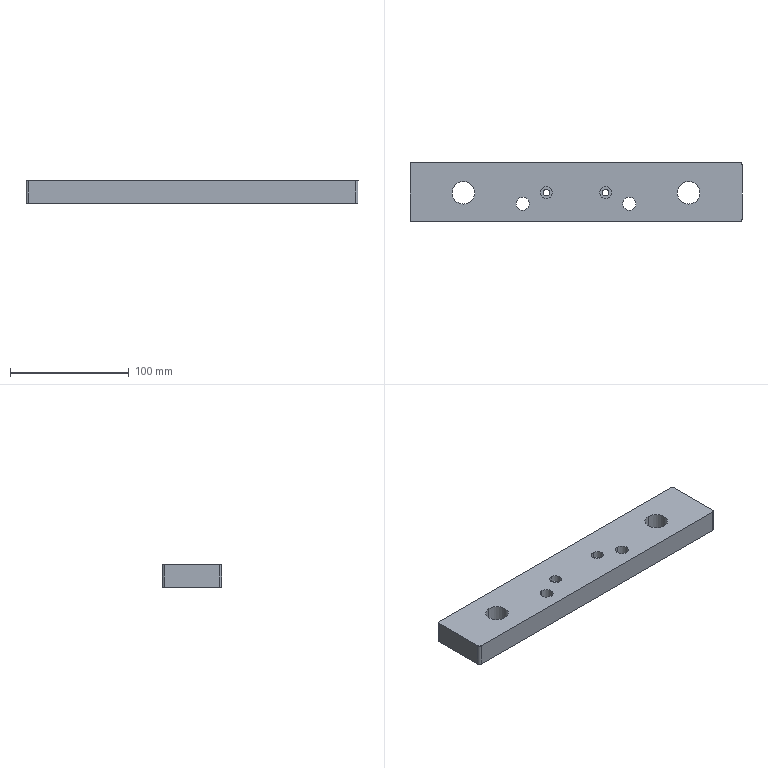Component | SolidWorks | 2SZT-2-001-3 | 1 solid | 33 faces | box 280 x 50 x 19.01 mm | volume 247242 mm3 | cylinder 20 | plane 13 | commonest cylinder face diameters 11 x4 10 x4 5.5 x4 19.02 x4 4 x4
build123d program:
from build123d import *

# Parameters (mm, degrees)
SKETCH1_W                                            = 280
SKETCH1_H                                            = 50
BOSS_EXTRUDE1_DEPTH                                  = 19
FILLET1_R                                            = 2
FILLET2_R                                            = 2
FILLET3_R                                            = 2
FILLET4_R                                            = 2
SKETCH11_W                                           = 62
SKETCH11_H                                           = 23
CUT_EXTRUDE2_DEPTH                                   = 2
F_10_0_10_DIAMETER_HOLE1_D                           = 19.02
F_10_0_10_DIAMETER_HOLE1_DEPTH                       = 70
F_10_0_10_DIAMETER_HOLE1_TIP                         = 5.714
HOLE_SIZE_ACCORDING_TO_THE_TYPE_OF_HEXAG_D           = 5.5
HOLE_SIZE_ACCORDING_TO_THE_TYPE_OF_HEXAG_CBORE_D     = 10
HOLE_SIZE_ACCORDING_TO_THE_TYPE_OF_HEXAG_CBORE_DEPTH = 5.7
F_11_0_11_DIAMETER_HOLE1_D                           = 11
F_11_0_11_DIAMETER_HOLE1_DEPTH                       = 20
F_11_0_11_DIAMETER_HOLE1_TIP                         = 3.305


with BuildPart() as part:
    # Sketch1 → Boss-Extrude1 (new body)
    with BuildSketch(Plane(origin=(0, 117.1, 0), x_dir=(-1, 0, 0), z_dir=(0, 1, 0))):
        with Locations((89.2, -92.53)):
            Rectangle(SKETCH1_W, SKETCH1_H)
    extrude(amount=-BOSS_EXTRUDE1_DEPTH)

    # Fillet1
    fillet1_edges = [part.edges().sort_by_distance(p)[0] for p in [
        (-229.2, 107.6, -67.53),
    ]]
    fillet(fillet1_edges, radius=FILLET1_R)

    # Fillet2
    fillet2_edges = [part.edges().sort_by_distance(p)[0] for p in [
        (-229.2, 107.6, -117.53),
    ]]
    fillet(fillet2_edges, radius=FILLET2_R)

    # Fillet3
    fillet3_edges = [part.edges().sort_by_distance(p)[0] for p in [
        (50.8, 107.6, -67.53),
    ]]
    fillet(fillet3_edges, radius=FILLET3_R)

    # Fillet4
    fillet4_edges = [part.edges().sort_by_distance(p)[0] for p in [
        (50.8, 107.6, -117.53),
    ]]
    fillet(fillet4_edges, radius=FILLET4_R)

    # Sketch11 → Cut-Extrude2 (cut)
    with BuildSketch(Plane(origin=(0, 117.1, 0), x_dir=(-1, 0, 0), z_dir=(0, 1, 0))):
        with Locations((89.2, -93.03)):
            Rectangle(SKETCH11_W, SKETCH11_H)
    extrude(amount=-CUT_EXTRUDE2_DEPTH, mode=Mode.SUBTRACT)

    # 10.0 _10_ Diameter Hole1
    with Locations(Plane.XZ.offset(-98.1)):
        with Locations((-184.2, -93.238), (5.8, -93.238)):
            Hole(F_10_0_10_DIAMETER_HOLE1_D / 2, depth=F_10_0_10_DIAMETER_HOLE1_DEPTH)
            with Locations((0, 0, -(F_10_0_10_DIAMETER_HOLE1_DEPTH + F_10_0_10_DIAMETER_HOLE1_TIP / 2))):  # 118° drill point
                Cone(0, F_10_0_10_DIAMETER_HOLE1_D / 2, F_10_0_10_DIAMETER_HOLE1_TIP, mode=Mode.SUBTRACT)

    # Hole Size according to the type of hexag (through all)
    with Locations(Plane.XZ.offset(-98.1)):
        with Locations((-114.2, -93.03), (-64.2, -93.03)):
            CounterBoreHole(HOLE_SIZE_ACCORDING_TO_THE_TYPE_OF_HEXAG_D / 2, HOLE_SIZE_ACCORDING_TO_THE_TYPE_OF_HEXAG_CBORE_D / 2, HOLE_SIZE_ACCORDING_TO_THE_TYPE_OF_HEXAG_CBORE_DEPTH)

    # 11.0 _11_ Diameter Hole1
    with Locations(Plane(origin=(0, 117.1, 0), x_dir=(1, 0, 0), z_dir=(0, 1, 0))):
        with Locations((-134.2, 102.43), (-44.2, 102.43)):
            Hole(F_11_0_11_DIAMETER_HOLE1_D / 2, depth=F_11_0_11_DIAMETER_HOLE1_DEPTH)
            with Locations((0, 0, -(F_11_0_11_DIAMETER_HOLE1_DEPTH + F_11_0_11_DIAMETER_HOLE1_TIP / 2))):  # 118° drill point
                Cone(0, F_11_0_11_DIAMETER_HOLE1_D / 2, F_11_0_11_DIAMETER_HOLE1_TIP, mode=Mode.SUBTRACT)


solid = part.part

# Placed as in the assembly
solid = solid.moved(Location((1044.465, 477.623, -197.096), (-90, 0, 0)))
STEP:
#1=CARTESIAN_POINT('',(35.837,14.555,-11.622));
#2=VERTEX_POINT('',#1);
#3=CARTESIAN_POINT('',(35.837,14.988,-11.622));
#4=VERTEX_POINT('',#3);
#5=CARTESIAN_POINT('',(35.837,14.771,-11.622));
#6=DIRECTION('',(-0.00002551,-0.,-1.));
#7=DIRECTION('',(0.,1.,0.));
#8=AXIS2_PLACEMENT_3D('',#5,#6,#7);
#9=CIRCLE('',#8,0.2165);
#10=EDGE_CURVE('',#2,#4,#9,.T.);
#11=ORIENTED_EDGE('',*,*,#10,.F.);
#12=CARTESIAN_POINT('',(35.837,14.555,-12.37));
#13=VERTEX_POINT('',#12);
#14=CARTESIAN_POINT('',(35.837,14.555,-12.37));
#15=DIRECTION('',(-0.00002551,-0.,-1.));
#16=VECTOR('',#15,39.37);
#17=LINE('',#14,#16);
#18=EDGE_CURVE('',#2,#13,#17,.T.);
#19=ORIENTED_EDGE('',*,*,#18,.T.);
#20=CARTESIAN_POINT('',(35.837,14.988,-12.37));
#21=VERTEX_POINT('',#20);
#22=CARTESIAN_POINT('',(35.837,14.771,-12.37));
#23=DIRECTION('',(-0.00002551,-0.,-1.));
#24=DIRECTION('',(0.,1.,0.));
#25=AXIS2_PLACEMENT_3D('',#22,#23,#24);
#26=CIRCLE('',#25,0.2165);
#27=EDGE_CURVE('',#13,#21,#26,.T.);
#28=ORIENTED_EDGE('',*,*,#27,.T.);
#29=CARTESIAN_POINT('',(35.837,14.988,-12.37));
#30=DIRECTION('',(-0.00002551,-0.,-1.));
#31=VECTOR('',#30,39.37);
#32=LINE('',#29,#31);
#33=EDGE_CURVE('',#4,#21,#32,.T.);
#34=ORIENTED_EDGE('',*,*,#33,.F.);
#35=EDGE_LOOP('',(#11,#19,#28,#34));
#36=FACE_OUTER_BOUND('',#35,.T.);
#37=CARTESIAN_POINT('',(35.837,14.771,-12.37));
#38=DIRECTION('',(-0.00002551,-0.,-1.));
#39=DIRECTION('',(0.,1.,0.));
#40=AXIS2_PLACEMENT_3D('',#37,#38,#39);
#41=CYLINDRICAL_SURFACE('',#40,0.2165);
#42=ADVANCED_FACE('',(#36),#41,.F.);
#43=CARTESIAN_POINT('',(39.381,14.555,-11.622));
#44=VERTEX_POINT('',#43);
#45=CARTESIAN_POINT('',(39.381,14.988,-11.622));
#46=VERTEX_POINT('',#45);
#47=CARTESIAN_POINT('',(39.381,14.771,-11.622));
#48=DIRECTION('',(-0.00002551,-0.,-1.));
#49=DIRECTION('',(0.,1.,0.));
#50=AXIS2_PLACEMENT_3D('',#47,#48,#49);
#51=CIRCLE('',#50,0.2165);
#52=EDGE_CURVE('',#44,#46,#51,.T.);
#53=ORIENTED_EDGE('',*,*,#52,.F.);
#54=CARTESIAN_POINT('',(39.381,14.555,-12.37));
#55=VERTEX_POINT('',#54);
#56=CARTESIAN_POINT('',(39.381,14.555,-12.37));
#57=DIRECTION('',(-0.00002551,-0.,-1.));
#58=VECTOR('',#57,39.37);
#59=LINE('',#56,#58);
#60=EDGE_CURVE('',#44,#55,#59,.T.);
#61=ORIENTED_EDGE('',*,*,#60,.T.);
#62=CARTESIAN_POINT('',(39.381,14.988,-12.37));
#63=VERTEX_POINT('',#62);
#64=CARTESIAN_POINT('',(39.381,14.771,-12.37));
#65=DIRECTION('',(-0.00002551,-0.,-1.));
#66=DIRECTION('',(0.,1.,0.));
#67=AXIS2_PLACEMENT_3D('',#64,#65,#66);
#68=CIRCLE('',#67,0.2165);
#69=EDGE_CURVE('',#55,#63,#68,.T.);
#70=ORIENTED_EDGE('',*,*,#69,.T.);
#71=CARTESIAN_POINT('',(39.381,14.988,-12.37));
#72=DIRECTION('',(-0.00002551,-0.,-1.));
#73=VECTOR('',#72,39.37);
#74=LINE('',#71,#73);
#75=EDGE_CURVE('',#46,#63,#74,.T.);
#76=ORIENTED_EDGE('',*,*,#75,.F.);
#77=EDGE_LOOP('',(#53,#61,#70,#76));
#78=FACE_OUTER_BOUND('',#77,.T.);
#79=CARTESIAN_POINT('',(39.381,14.771,-12.37));
#80=DIRECTION('',(-0.00002551,-0.,-1.));
#81=DIRECTION('',(0.,1.,0.));
#82=AXIS2_PLACEMENT_3D('',#79,#80,#81);
#83=CYLINDRICAL_SURFACE('',#82,0.2165);
#84=ADVANCED_FACE('',(#78),#83,.F.);
#85=CARTESIAN_POINT('',(36.625,15.338,-11.846));
#86=VERTEX_POINT('',#85);
#87=CARTESIAN_POINT('',(36.625,14.945,-11.846));
#88=VERTEX_POINT('',#87);
#89=CARTESIAN_POINT('',(36.625,15.141,-11.846));
#90=DIRECTION('',(0.00002551,0.,1.));
#91=DIRECTION('',(0.,-1.,0.));
#92=AXIS2_PLACEMENT_3D('',#89,#90,#91);
#93=CIRCLE('',#92,0.1969);
#94=EDGE_CURVE('',#86,#88,#93,.T.);
#95=ORIENTED_EDGE('',*,*,#94,.F.);
#96=CARTESIAN_POINT('',(36.625,15.338,-11.622));
#97=VERTEX_POINT('',#96);
#98=CARTESIAN_POINT('',(36.625,15.338,-11.622));
#99=DIRECTION('',(0.00002551,0.,1.));
#100=VECTOR('',#99,39.37);
#101=LINE('',#98,#100);
#102=EDGE_CURVE('',#86,#97,#101,.T.);
#103=ORIENTED_EDGE('',*,*,#102,.T.);
#104=CARTESIAN_POINT('',(36.625,14.945,-11.622));
#105=VERTEX_POINT('',#104);
#106=CARTESIAN_POINT('',(36.625,15.141,-11.622));
#107=DIRECTION('',(0.00002551,0.,1.));
#108=DIRECTION('',(0.,-1.,0.));
#109=AXIS2_PLACEMENT_3D('',#106,#107,#108);
#110=CIRCLE('',#109,0.1969);
#111=EDGE_CURVE('',#97,#105,#110,.T.);
#112=ORIENTED_EDGE('',*,*,#111,.T.);
#113=CARTESIAN_POINT('',(36.625,14.945,-11.622));
#114=DIRECTION('',(0.00002551,0.,1.));
#115=VECTOR('',#114,39.37);
#116=LINE('',#113,#115);
#117=EDGE_CURVE('',#88,#105,#116,.T.);
#118=ORIENTED_EDGE('',*,*,#117,.F.);
#119=EDGE_LOOP('',(#95,#103,#112,#118));
#120=FACE_OUTER_BOUND('',#119,.T.);
#121=CARTESIAN_POINT('',(36.625,15.141,-11.622));
#122=DIRECTION('',(0.00002551,0.,1.));
#123=DIRECTION('',(0.,-1.,0.));
#124=AXIS2_PLACEMENT_3D('',#121,#122,#123);
#125=CYLINDRICAL_SURFACE('',#124,0.1969);
#126=ADVANCED_FACE('',(#120),#125,.F.);
#127=CARTESIAN_POINT('',(36.625,15.033,-12.291));
#128=VERTEX_POINT('',#127);
#129=CARTESIAN_POINT('',(36.625,15.25,-12.291));
#130=VERTEX_POINT('',#129);
#131=CARTESIAN_POINT('',(36.625,15.141,-12.291));
#132=DIRECTION('',(-0.00002551,-0.,-1.));
#133=DIRECTION('',(0.,1.,0.));
#134=AXIS2_PLACEMENT_3D('',#131,#132,#133);
#135=CIRCLE('',#134,0.1083);
#136=EDGE_CURVE('',#128,#130,#135,.T.);
#137=ORIENTED_EDGE('',*,*,#136,.T.);
#138=CARTESIAN_POINT('',(36.625,15.25,-11.846));
#139=VERTEX_POINT('',#138);
#140=CARTESIAN_POINT('',(36.625,15.25,-11.622));
#141=DIRECTION('',(0.00002551,0.,1.));
#142=VECTOR('',#141,39.37);
#143=LINE('',#140,#142);
#144=EDGE_CURVE('',#130,#139,#143,.T.);
#145=ORIENTED_EDGE('',*,*,#144,.T.);
#146=CARTESIAN_POINT('',(36.625,15.033,-11.846));
#147=VERTEX_POINT('',#146);
#148=CARTESIAN_POINT('',(36.625,15.141,-11.846));
#149=DIRECTION('',(0.00002551,0.,1.));
#150=DIRECTION('',(0.,-1.,0.));
#151=AXIS2_PLACEMENT_3D('',#148,#149,#150);
#152=CIRCLE('',#151,0.1083);
#153=EDGE_CURVE('',#139,#147,#152,.T.);
#154=ORIENTED_EDGE('',*,*,#153,.T.);
#155=CARTESIAN_POINT('',(36.625,15.033,-11.622));
#156=DIRECTION('',(0.00002551,0.,1.));
#157=VECTOR('',#156,39.37);
#158=LINE('',#155,#157);
#159=EDGE_CURVE('',#128,#147,#158,.T.);
#160=ORIENTED_EDGE('',*,*,#159,.F.);
#161=EDGE_LOOP('',(#137,#145,#154,#160));
#162=FACE_OUTER_BOUND('',#161,.T.);
#163=CARTESIAN_POINT('',(36.625,15.141,-11.622));
#164=DIRECTION('',(0.00002551,0.,1.));
#165=DIRECTION('',(0.,-1.,0.));
#166=AXIS2_PLACEMENT_3D('',#163,#164,#165);
#167=CYLINDRICAL_SURFACE('',#166,0.1083);
#168=ADVANCED_FACE('',(#162),#167,.F.);
#169=CARTESIAN_POINT('',(38.593,15.338,-11.846));
#170=VERTEX_POINT('',#169);
#171=CARTESIAN_POINT('',(38.593,14.945,-11.846));
#172=VERTEX_POINT('',#171);
#173=CARTESIAN_POINT('',(38.593,15.141,-11.846));
#174=DIRECTION('',(0.00002551,0.,1.));
#175=DIRECTION('',(0.,-1.,0.));
#176=AXIS2_PLACEMENT_3D('',#173,#174,#175);
#177=CIRCLE('',#176,0.1969);
#178=EDGE_CURVE('',#170,#172,#177,.T.);
#179=ORIENTED_EDGE('',*,*,#178,.F.);
#180=CARTESIAN_POINT('',(38.593,15.338,-11.622));
#181=VERTEX_POINT('',#180);
#182=CARTESIAN_POINT('',(38.593,15.338,-11.622));
#183=DIRECTION('',(0.00002551,0.,1.));
#184=VECTOR('',#183,39.37);
#185=LINE('',#182,#184);
#186=EDGE_CURVE('',#170,#181,#185,.T.);
#187=ORIENTED_EDGE('',*,*,#186,.T.);
#188=CARTESIAN_POINT('',(38.593,14.945,-11.622));
#189=VERTEX_POINT('',#188);
#190=CARTESIAN_POINT('',(38.593,15.141,-11.622));
#191=DIRECTION('',(0.00002551,0.,1.));
#192=DIRECTION('',(0.,-1.,0.));
#193=AXIS2_PLACEMENT_3D('',#190,#191,#192);
#194=CIRCLE('',#193,0.1969);
#195=EDGE_CURVE('',#181,#189,#194,.T.);
#196=ORIENTED_EDGE('',*,*,#195,.T.);
#197=CARTESIAN_POINT('',(38.593,14.945,-11.622));
#198=DIRECTION('',(0.00002551,0.,1.));
#199=VECTOR('',#198,39.37);
#200=LINE('',#197,#199);
#201=EDGE_CURVE('',#172,#189,#200,.T.);
#202=ORIENTED_EDGE('',*,*,#201,.F.);
#203=EDGE_LOOP('',(#179,#187,#196,#202));
#204=FACE_OUTER_BOUND('',#203,.T.);
#205=CARTESIAN_POINT('',(38.593,15.141,-11.622));
#206=DIRECTION('',(0.00002551,0.,1.));
#207=DIRECTION('',(0.,-1.,0.));
#208=AXIS2_PLACEMENT_3D('',#205,#206,#207);
#209=CYLINDRICAL_SURFACE('',#208,0.1969);
#210=ADVANCED_FACE('',(#204),#209,.F.);
#211=CARTESIAN_POINT('',(38.593,15.033,-12.291));
#212=VERTEX_POINT('',#211);
#213=CARTESIAN_POINT('',(38.593,15.25,-12.291));
#214=VERTEX_POINT('',#213);
#215=CARTESIAN_POINT('',(38.593,15.141,-12.291));
#216=DIRECTION('',(-0.00002551,-0.,-1.));
#217=DIRECTION('',(0.,1.,0.));
#218=AXIS2_PLACEMENT_3D('',#215,#216,#217);
#219=CIRCLE('',#218,0.1083);
#220=EDGE_CURVE('',#212,#214,#219,.T.);
#221=ORIENTED_EDGE('',*,*,#220,.T.);
#222=CARTESIAN_POINT('',(38.593,15.25,-11.846));
#223=VERTEX_POINT('',#222);
#224=CARTESIAN_POINT('',(38.593,15.25,-11.622));
#225=DIRECTION('',(0.00002551,0.,1.));
#226=VECTOR('',#225,39.37);
#227=LINE('',#224,#226);
#228=EDGE_CURVE('',#214,#223,#227,.T.);
#229=ORIENTED_EDGE('',*,*,#228,.T.);
#230=CARTESIAN_POINT('',(38.593,15.033,-11.846));
#231=VERTEX_POINT('',#230);
#232=CARTESIAN_POINT('',(38.593,15.141,-11.846));
#233=DIRECTION('',(0.00002551,0.,1.));
#234=DIRECTION('',(0.,-1.,0.));
#235=AXIS2_PLACEMENT_3D('',#232,#233,#234);
#236=CIRCLE('',#235,0.1083);
#237=EDGE_CURVE('',#223,#231,#236,.T.);
#238=ORIENTED_EDGE('',*,*,#237,.T.);
#239=CARTESIAN_POINT('',(38.593,15.033,-11.622));
#240=DIRECTION('',(0.00002551,0.,1.));
#241=VECTOR('',#240,39.37);
#242=LINE('',#239,#241);
#243=EDGE_CURVE('',#212,#231,#242,.T.);
#244=ORIENTED_EDGE('',*,*,#243,.F.);
#245=EDGE_LOOP('',(#221,#229,#238,#244));
#246=FACE_OUTER_BOUND('',#245,.T.);
#247=CARTESIAN_POINT('',(38.593,15.141,-11.622));
#248=DIRECTION('',(0.00002551,0.,1.));
#249=DIRECTION('',(0.,-1.,0.));
#250=AXIS2_PLACEMENT_3D('',#247,#248,#249);
#251=CYLINDRICAL_SURFACE('',#250,0.1083);
#252=ADVANCED_FACE('',(#246),#251,.F.);
#253=CARTESIAN_POINT('',(33.869,14.759,-12.37));
#254=VERTEX_POINT('',#253);
#255=CARTESIAN_POINT('',(33.869,15.508,-12.37));
#256=VERTEX_POINT('',#255);
#257=CARTESIAN_POINT('',(33.869,15.133,-12.37));
#258=DIRECTION('',(-0.00002551,-0.,-1.));
#259=DIRECTION('',(0.,1.,0.));
#260=AXIS2_PLACEMENT_3D('',#257,#258,#259);
#261=CIRCLE('',#260,0.3744);
#262=EDGE_CURVE('',#254,#256,#261,.T.);
#263=ORIENTED_EDGE('',*,*,#262,.T.);
#264=CARTESIAN_POINT('',(33.869,15.508,-11.622));
#265=VERTEX_POINT('',#264);
#266=CARTESIAN_POINT('',(33.869,15.508,-11.622));
#267=DIRECTION('',(0.00002551,0.,1.));
#268=VECTOR('',#267,39.37);
#269=LINE('',#266,#268);
#270=EDGE_CURVE('',#256,#265,#269,.T.);
#271=ORIENTED_EDGE('',*,*,#270,.T.);
#272=CARTESIAN_POINT('',(33.869,14.759,-11.622));
#273=VERTEX_POINT('',#272);
#274=CARTESIAN_POINT('',(33.869,15.133,-11.622));
#275=DIRECTION('',(0.00002551,0.,1.));
#276=DIRECTION('',(0.,-1.,0.));
#277=AXIS2_PLACEMENT_3D('',#274,#275,#276);
#278=CIRCLE('',#277,0.3744);
#279=EDGE_CURVE('',#265,#273,#278,.T.);
#280=ORIENTED_EDGE('',*,*,#279,.T.);
#281=CARTESIAN_POINT('',(33.869,14.759,-11.622));
#282=DIRECTION('',(0.00002551,0.,1.));
#283=VECTOR('',#282,39.37);
#284=LINE('',#281,#283);
#285=EDGE_CURVE('',#254,#273,#284,.T.);
#286=ORIENTED_EDGE('',*,*,#285,.F.);
#287=EDGE_LOOP('',(#263,#271,#280,#286));
#288=FACE_OUTER_BOUND('',#287,.T.);
#289=CARTESIAN_POINT('',(33.869,15.133,-11.622));
#290=DIRECTION('',(0.00002551,0.,1.));
#291=DIRECTION('',(0.,-1.,0.));
#292=AXIS2_PLACEMENT_3D('',#289,#290,#291);
#293=CYLINDRICAL_SURFACE('',#292,0.3744);
#294=ADVANCED_FACE('',(#288),#293,.F.);
#295=CARTESIAN_POINT('',(41.349,14.759,-12.37));
#296=VERTEX_POINT('',#295);
#297=CARTESIAN_POINT('',(41.349,15.508,-12.37));
#298=VERTEX_POINT('',#297);
#299=CARTESIAN_POINT('',(41.349,15.133,-12.37));
#300=DIRECTION('',(-0.00002551,-0.,-1.));
#301=DIRECTION('',(0.,1.,0.));
#302=AXIS2_PLACEMENT_3D('',#299,#300,#301);
#303=CIRCLE('',#302,0.3744);
#304=EDGE_CURVE('',#296,#298,#303,.T.);
#305=ORIENTED_EDGE('',*,*,#304,.T.);
#306=CARTESIAN_POINT('',(41.349,15.508,-11.622));
#307=VERTEX_POINT('',#306);
#308=CARTESIAN_POINT('',(41.349,15.508,-11.622));
#309=DIRECTION('',(0.00002551,0.,1.));
#310=VECTOR('',#309,39.37);
#311=LINE('',#308,#310);
#312=EDGE_CURVE('',#298,#307,#311,.T.);
#313=ORIENTED_EDGE('',*,*,#312,.T.);
#314=CARTESIAN_POINT('',(41.349,14.759,-11.622));
#315=VERTEX_POINT('',#314);
#316=CARTESIAN_POINT('',(41.349,15.133,-11.622));
#317=DIRECTION('',(0.00002551,0.,1.));
#318=DIRECTION('',(0.,-1.,0.));
#319=AXIS2_PLACEMENT_3D('',#316,#317,#318);
#320=CIRCLE('',#319,0.3744);
#321=EDGE_CURVE('',#307,#315,#320,.T.);
#322=ORIENTED_EDGE('',*,*,#321,.T.);
#323=CARTESIAN_POINT('',(41.349,14.759,-11.622));
#324=DIRECTION('',(0.00002551,0.,1.));
#325=VECTOR('',#324,39.37);
#326=LINE('',#323,#325);
#327=EDGE_CURVE('',#296,#315,#326,.T.);
#328=ORIENTED_EDGE('',*,*,#327,.F.);
#329=EDGE_LOOP('',(#305,#313,#322,#328));
#330=FACE_OUTER_BOUND('',#329,.T.);
#331=CARTESIAN_POINT('',(41.349,15.133,-11.622));
#332=DIRECTION('',(0.00002551,0.,1.));
#333=DIRECTION('',(0.,-1.,0.));
#334=AXIS2_PLACEMENT_3D('',#331,#332,#333);
#335=CYLINDRICAL_SURFACE('',#334,0.3744);
#336=ADVANCED_FACE('',(#330),#335,.F.);
#337=CARTESIAN_POINT('',(43.121,16.067,-11.622));
#338=VERTEX_POINT('',#337);
#339=CARTESIAN_POINT('',(43.121,14.256,-11.622));
#340=VERTEX_POINT('',#339);
#341=CARTESIAN_POINT('',(43.121,16.145,-11.622));
#342=DIRECTION('',(-0.,-1.,0.));
#343=VECTOR('',#342,39.37);
#344=LINE('',#341,#343);
#345=EDGE_CURVE('',#338,#340,#344,.T.);
#346=ORIENTED_EDGE('',*,*,#345,.T.);
#347=CARTESIAN_POINT('',(43.121,14.256,-12.37));
#348=VERTEX_POINT('',#347);
#349=CARTESIAN_POINT('',(43.121,14.256,-11.622));
#350=DIRECTION('',(-0.00002551,-0.,-1.));
#351=VECTOR('',#350,39.37);
#352=LINE('',#349,#351);
#353=EDGE_CURVE('',#340,#348,#352,.T.);
#354=ORIENTED_EDGE('',*,*,#353,.T.);
#355=CARTESIAN_POINT('',(43.121,16.067,-12.37));
#356=VERTEX_POINT('',#355);
#357=CARTESIAN_POINT('',(43.121,16.145,-12.37));
#358=DIRECTION('',(-0.,-1.,0.));
#359=VECTOR('',#358,39.37);
#360=LINE('',#357,#359);
#361=EDGE_CURVE('',#356,#348,#360,.T.);
#362=ORIENTED_EDGE('',*,*,#361,.F.);
#363=CARTESIAN_POINT('',(43.121,16.067,-11.622));
#364=DIRECTION('',(0.00002551,0.,1.));
#365=VECTOR('',#364,39.37);
#366=LINE('',#363,#365);
#367=EDGE_CURVE('',#356,#338,#366,.T.);
#368=ORIENTED_EDGE('',*,*,#367,.T.);
#369=EDGE_LOOP('',(#346,#354,#362,#368));
#370=FACE_OUTER_BOUND('',#369,.T.);
#371=CARTESIAN_POINT('',(43.121,16.145,-11.622));
#372=DIRECTION('',(1.,-0.,-0.00002551));
#373=DIRECTION('',(-0.,-1.,0.));
#374=AXIS2_PLACEMENT_3D('',#371,#372,#373);
#375=PLANE('',#374);
#376=ADVANCED_FACE('',(#370),#375,.T.);
#377=CARTESIAN_POINT('',(32.176,16.145,-11.622));
#378=VERTEX_POINT('',#377);
#379=CARTESIAN_POINT('',(43.042,16.145,-11.622));
#380=VERTEX_POINT('',#379);
#381=CARTESIAN_POINT('',(32.097,16.145,-11.622));
#382=DIRECTION('',(1.,-0.,-0.00002551));
#383=VECTOR('',#382,39.37);
#384=LINE('',#381,#383);
#385=EDGE_CURVE('',#378,#380,#384,.T.);
#386=ORIENTED_EDGE('',*,*,#385,.T.);
#387=CARTESIAN_POINT('',(43.042,16.145,-12.37));
#388=VERTEX_POINT('',#387);
#389=CARTESIAN_POINT('',(43.042,16.145,-11.622));
#390=DIRECTION('',(-0.00002551,-0.,-1.));
#391=VECTOR('',#390,39.37);
#392=LINE('',#389,#391);
#393=EDGE_CURVE('',#380,#388,#392,.T.);
#394=ORIENTED_EDGE('',*,*,#393,.T.);
#395=CARTESIAN_POINT('',(32.176,16.145,-12.37));
#396=VERTEX_POINT('',#395);
#397=CARTESIAN_POINT('',(32.097,16.145,-12.37));
#398=DIRECTION('',(1.,-0.,-0.00002551));
#399=VECTOR('',#398,39.37);
#400=LINE('',#397,#399);
#401=EDGE_CURVE('',#396,#388,#400,.T.);
#402=ORIENTED_EDGE('',*,*,#401,.F.);
#403=CARTESIAN_POINT('',(32.176,16.145,-11.622));
#404=DIRECTION('',(0.00002551,0.,1.));
#405=VECTOR('',#404,39.37);
#406=LINE('',#403,#405);
#407=EDGE_CURVE('',#396,#378,#406,.T.);
#408=ORIENTED_EDGE('',*,*,#407,.T.);
#409=EDGE_LOOP('',(#386,#394,#402,#408));
#410=FACE_OUTER_BOUND('',#409,.T.);
#411=CARTESIAN_POINT('',(32.097,16.145,-11.622));
#412=DIRECTION('',(0.,1.,-0.));
#413=DIRECTION('',(1.,-0.,-0.00002551));
#414=AXIS2_PLACEMENT_3D('',#411,#412,#413);
#415=PLANE('',#414);
#416=ADVANCED_FACE('',(#410),#415,.T.);
#417=CARTESIAN_POINT('',(32.097,14.256,-12.37));
#418=VERTEX_POINT('',#417);
#419=CARTESIAN_POINT('',(32.097,16.067,-12.37));
#420=VERTEX_POINT('',#419);
#421=CARTESIAN_POINT('',(32.097,14.177,-12.37));
#422=DIRECTION('',(0.,1.,-0.));
#423=VECTOR('',#422,39.37);
#424=LINE('',#421,#423);
#425=EDGE_CURVE('',#418,#420,#424,.T.);
#426=ORIENTED_EDGE('',*,*,#425,.F.);
#427=CARTESIAN_POINT('',(32.097,14.256,-11.622));
#428=VERTEX_POINT('',#427);
#429=CARTESIAN_POINT('',(32.097,14.256,-11.622));
#430=DIRECTION('',(0.00002551,0.,1.));
#431=VECTOR('',#430,39.37);
#432=LINE('',#429,#431);
#433=EDGE_CURVE('',#418,#428,#432,.T.);
#434=ORIENTED_EDGE('',*,*,#433,.T.);
#435=CARTESIAN_POINT('',(32.097,16.067,-11.622));
#436=VERTEX_POINT('',#435);
#437=CARTESIAN_POINT('',(32.097,14.177,-11.622));
#438=DIRECTION('',(0.,1.,-0.));
#439=VECTOR('',#438,39.37);
#440=LINE('',#437,#439);
#441=EDGE_CURVE('',#428,#436,#440,.T.);
#442=ORIENTED_EDGE('',*,*,#441,.T.);
#443=CARTESIAN_POINT('',(32.097,16.067,-11.622));
#444=DIRECTION('',(-0.00002551,-0.,-1.));
#445=VECTOR('',#444,39.37);
#446=LINE('',#443,#445);
#447=EDGE_CURVE('',#436,#420,#446,.T.);
#448=ORIENTED_EDGE('',*,*,#447,.T.);
#449=EDGE_LOOP('',(#426,#434,#442,#448));
#450=FACE_OUTER_BOUND('',#449,.T.);
#451=CARTESIAN_POINT('',(32.097,14.177,-11.622));
#452=DIRECTION('',(-1.,0.,0.00002551));
#453=DIRECTION('',(0.,1.,-0.));
#454=AXIS2_PLACEMENT_3D('',#451,#452,#453);
#455=PLANE('',#454);
#456=ADVANCED_FACE('',(#450),#455,.T.);
#457=CARTESIAN_POINT('',(43.042,14.177,-12.37));
#458=VERTEX_POINT('',#457);
#459=CARTESIAN_POINT('',(32.176,14.177,-12.37));
#460=VERTEX_POINT('',#459);
#461=CARTESIAN_POINT('',(43.121,14.177,-12.37));
#462=DIRECTION('',(-1.,0.,0.00002551));
#463=VECTOR('',#462,39.37);
#464=LINE('',#461,#463);
#465=EDGE_CURVE('',#458,#460,#464,.T.);
#466=ORIENTED_EDGE('',*,*,#465,.F.);
#467=CARTESIAN_POINT('',(43.042,14.177,-11.622));
#468=VERTEX_POINT('',#467);
#469=CARTESIAN_POINT('',(43.042,14.177,-11.622));
#470=DIRECTION('',(0.00002551,0.,1.));
#471=VECTOR('',#470,39.37);
#472=LINE('',#469,#471);
#473=EDGE_CURVE('',#458,#468,#472,.T.);
#474=ORIENTED_EDGE('',*,*,#473,.T.);
#475=CARTESIAN_POINT('',(32.176,14.177,-11.622));
#476=VERTEX_POINT('',#475);
#477=CARTESIAN_POINT('',(43.121,14.177,-11.622));
#478=DIRECTION('',(-1.,0.,0.00002551));
#479=VECTOR('',#478,39.37);
#480=LINE('',#477,#479);
#481=EDGE_CURVE('',#468,#476,#480,.T.);
#482=ORIENTED_EDGE('',*,*,#481,.T.);
#483=CARTESIAN_POINT('',(32.176,14.177,-11.622));
#484=DIRECTION('',(-0.00002551,-0.,-1.));
#485=VECTOR('',#484,39.37);
#486=LINE('',#483,#485);
#487=EDGE_CURVE('',#476,#460,#486,.T.);
#488=ORIENTED_EDGE('',*,*,#487,.T.);
#489=EDGE_LOOP('',(#466,#474,#482,#488));
#490=FACE_OUTER_BOUND('',#489,.T.);
#491=CARTESIAN_POINT('',(43.121,14.177,-11.622));
#492=DIRECTION('',(-0.,-1.,0.));
#493=DIRECTION('',(-1.,0.,0.00002551));
#494=AXIS2_PLACEMENT_3D('',#491,#492,#493);
#495=PLANE('',#494);
#496=ADVANCED_FACE('',(#490),#495,.T.);
#497=CARTESIAN_POINT('',(35.837,14.771,-11.622));
#498=DIRECTION('',(-0.00002551,-0.,-1.));
#499=DIRECTION('',(0.,1.,0.));
#500=AXIS2_PLACEMENT_3D('',#497,#498,#499);
#501=CIRCLE('',#500,0.2165);
#502=EDGE_CURVE('',#4,#2,#501,.T.);
#503=ORIENTED_EDGE('',*,*,#502,.T.);
#504=ORIENTED_EDGE('',*,*,#10,.T.);
#505=EDGE_LOOP('',(#503,#504));
#506=FACE_BOUND('',#505,.T.);
#507=CARTESIAN_POINT('',(39.381,14.771,-11.622));
#508=DIRECTION('',(-0.00002551,-0.,-1.));
#509=DIRECTION('',(0.,1.,0.));
#510=AXIS2_PLACEMENT_3D('',#507,#508,#509);
#511=CIRCLE('',#510,0.2165);
#512=EDGE_CURVE('',#46,#44,#511,.T.);
#513=ORIENTED_EDGE('',*,*,#512,.T.);
#514=ORIENTED_EDGE('',*,*,#52,.T.);
#515=EDGE_LOOP('',(#513,#514));
#516=FACE_BOUND('',#515,.T.);
#517=CARTESIAN_POINT('',(36.625,15.141,-11.622));
#518=DIRECTION('',(0.00002551,0.,1.));
#519=DIRECTION('',(0.,-1.,0.));
#520=AXIS2_PLACEMENT_3D('',#517,#518,#519);
#521=CIRCLE('',#520,0.1969);
#522=EDGE_CURVE('',#105,#97,#521,.T.);
#523=ORIENTED_EDGE('',*,*,#522,.F.);
#524=ORIENTED_EDGE('',*,*,#111,.F.);
#525=EDGE_LOOP('',(#523,#524));
#526=FACE_BOUND('',#525,.T.);
#527=CARTESIAN_POINT('',(38.593,15.141,-11.622));
#528=DIRECTION('',(0.00002551,0.,1.));
#529=DIRECTION('',(0.,-1.,0.));
#530=AXIS2_PLACEMENT_3D('',#527,#528,#529);
#531=CIRCLE('',#530,0.1969);
#532=EDGE_CURVE('',#189,#181,#531,.T.);
#533=ORIENTED_EDGE('',*,*,#532,.F.);
#534=ORIENTED_EDGE('',*,*,#195,.F.);
#535=EDGE_LOOP('',(#533,#534));
#536=FACE_BOUND('',#535,.T.);
#537=CARTESIAN_POINT('',(33.869,15.133,-11.622));
#538=DIRECTION('',(0.00002551,0.,1.));
#539=DIRECTION('',(0.,-1.,0.));
#540=AXIS2_PLACEMENT_3D('',#537,#538,#539);
#541=CIRCLE('',#540,0.3744);
#542=EDGE_CURVE('',#273,#265,#541,.T.);
#543=ORIENTED_EDGE('',*,*,#542,.F.);
#544=ORIENTED_EDGE('',*,*,#279,.F.);
#545=EDGE_LOOP('',(#543,#544));
#546=FACE_BOUND('',#545,.T.);
#547=CARTESIAN_POINT('',(41.349,15.133,-11.622));
#548=DIRECTION('',(0.00002551,0.,1.));
#549=DIRECTION('',(0.,-1.,0.));
#550=AXIS2_PLACEMENT_3D('',#547,#548,#549);
#551=CIRCLE('',#550,0.3744);
#552=EDGE_CURVE('',#315,#307,#551,.T.);
#553=ORIENTED_EDGE('',*,*,#552,.F.);
#554=ORIENTED_EDGE('',*,*,#321,.F.);
#555=EDGE_LOOP('',(#553,#554));
#556=FACE_BOUND('',#555,.T.);
#557=ORIENTED_EDGE('',*,*,#481,.F.);
#558=CARTESIAN_POINT('',(43.042,14.256,-11.622));
#559=DIRECTION('',(0.00002551,0.,1.));
#560=DIRECTION('',(0.,1.,0.));
#561=AXIS2_PLACEMENT_3D('',#558,#559,#560);
#562=CIRCLE('',#561,0.07874);
#563=EDGE_CURVE('',#468,#340,#562,.T.);
#564=ORIENTED_EDGE('',*,*,#563,.T.);
#565=ORIENTED_EDGE('',*,*,#345,.F.);
#566=CARTESIAN_POINT('',(43.042,16.067,-11.622));
#567=DIRECTION('',(0.00002551,0.,1.));
#568=DIRECTION('',(0.,1.,0.));
#569=AXIS2_PLACEMENT_3D('',#566,#567,#568);
#570=CIRCLE('',#569,0.07874);
#571=EDGE_CURVE('',#338,#380,#570,.T.);
#572=ORIENTED_EDGE('',*,*,#571,.T.);
#573=ORIENTED_EDGE('',*,*,#385,.F.);
#574=CARTESIAN_POINT('',(32.176,16.067,-11.622));
#575=DIRECTION('',(0.00002551,0.,1.));
#576=DIRECTION('',(0.,1.,0.));
#577=AXIS2_PLACEMENT_3D('',#574,#575,#576);
#578=CIRCLE('',#577,0.07874);
#579=EDGE_CURVE('',#378,#436,#578,.T.);
#580=ORIENTED_EDGE('',*,*,#579,.T.);
#581=ORIENTED_EDGE('',*,*,#441,.F.);
#582=CARTESIAN_POINT('',(32.176,14.256,-11.622));
#583=DIRECTION('',(0.00002551,0.,1.));
#584=DIRECTION('',(0.,1.,0.));
#585=AXIS2_PLACEMENT_3D('',#582,#583,#584);
#586=CIRCLE('',#585,0.07874);
#587=EDGE_CURVE('',#428,#476,#586,.T.);
#588=ORIENTED_EDGE('',*,*,#587,.T.);
#589=EDGE_LOOP('',(#557,#564,#565,#572,#573,#580,#581,#588));
#590=FACE_OUTER_BOUND('',#589,.T.);
#591=CARTESIAN_POINT('',(43.121,14.177,-11.622));
#592=DIRECTION('',(-0.00002551,-0.,-1.));
#593=DIRECTION('',(0.,1.,-0.));
#594=AXIS2_PLACEMENT_3D('',#591,#592,#593);
#595=PLANE('',#594);
#596=ADVANCED_FACE('',(#506,#516,#526,#536,#546,#556,#590),#595,.F.);
#597=CARTESIAN_POINT('',(35.837,14.771,-12.37));
#598=DIRECTION('',(-0.00002551,-0.,-1.));
#599=DIRECTION('',(0.,1.,0.));
#600=AXIS2_PLACEMENT_3D('',#597,#598,#599);
#601=CIRCLE('',#600,0.2165);
#602=EDGE_CURVE('',#21,#13,#601,.T.);
#603=ORIENTED_EDGE('',*,*,#602,.F.);
#604=ORIENTED_EDGE('',*,*,#27,.F.);
#605=EDGE_LOOP('',(#603,#604));
#606=FACE_BOUND('',#605,.T.);
#607=CARTESIAN_POINT('',(39.381,14.771,-12.37));
#608=DIRECTION('',(-0.00002551,-0.,-1.));
#609=DIRECTION('',(0.,1.,0.));
#610=AXIS2_PLACEMENT_3D('',#607,#608,#609);
#611=CIRCLE('',#610,0.2165);
#612=EDGE_CURVE('',#63,#55,#611,.T.);
#613=ORIENTED_EDGE('',*,*,#612,.F.);
#614=ORIENTED_EDGE('',*,*,#69,.F.);
#615=EDGE_LOOP('',(#613,#614));
#616=FACE_BOUND('',#615,.T.);
#617=ORIENTED_EDGE('',*,*,#262,.F.);
#618=CARTESIAN_POINT('',(33.869,15.133,-12.37));
#619=DIRECTION('',(-0.00002551,-0.,-1.));
#620=DIRECTION('',(0.,1.,0.));
#621=AXIS2_PLACEMENT_3D('',#618,#619,#620);
#622=CIRCLE('',#621,0.3744);
#623=EDGE_CURVE('',#256,#254,#622,.T.);
#624=ORIENTED_EDGE('',*,*,#623,.F.);
#625=EDGE_LOOP('',(#617,#624));
#626=FACE_BOUND('',#625,.T.);
#627=ORIENTED_EDGE('',*,*,#304,.F.);
#628=CARTESIAN_POINT('',(41.349,15.133,-12.37));
#629=DIRECTION('',(-0.00002551,-0.,-1.));
#630=DIRECTION('',(0.,1.,0.));
#631=AXIS2_PLACEMENT_3D('',#628,#629,#630);
#632=CIRCLE('',#631,0.3744);
#633=EDGE_CURVE('',#298,#296,#632,.T.);
#634=ORIENTED_EDGE('',*,*,#633,.F.);
#635=EDGE_LOOP('',(#627,#634));
#636=FACE_BOUND('',#635,.T.);
#637=CARTESIAN_POINT('',(36.388,14.689,-12.37));
#638=VERTEX_POINT('',#637);
#639=CARTESIAN_POINT('',(36.388,15.594,-12.37));
#640=VERTEX_POINT('',#639);
#641=CARTESIAN_POINT('',(36.388,14.689,-12.37));
#642=DIRECTION('',(0.,1.,-0.));
#643=VECTOR('',#642,39.37);
#644=LINE('',#641,#643);
#645=EDGE_CURVE('',#638,#640,#644,.T.);
#646=ORIENTED_EDGE('',*,*,#645,.F.);
#647=CARTESIAN_POINT('',(38.829,14.689,-12.37));
#648=VERTEX_POINT('',#647);
#649=CARTESIAN_POINT('',(36.388,14.689,-12.37));
#650=DIRECTION('',(-1.,0.,0.00002551));
#651=VECTOR('',#650,39.37);
#652=LINE('',#649,#651);
#653=EDGE_CURVE('',#648,#638,#652,.T.);
#654=ORIENTED_EDGE('',*,*,#653,.F.);
#655=CARTESIAN_POINT('',(38.829,15.594,-12.37));
#656=VERTEX_POINT('',#655);
#657=CARTESIAN_POINT('',(38.829,14.689,-12.37));
#658=DIRECTION('',(-0.,-1.,0.));
#659=VECTOR('',#658,39.37);
#660=LINE('',#657,#659);
#661=EDGE_CURVE('',#656,#648,#660,.T.);
#662=ORIENTED_EDGE('',*,*,#661,.F.);
#663=CARTESIAN_POINT('',(36.388,15.594,-12.37));
#664=DIRECTION('',(1.,-0.,-0.00002551));
#665=VECTOR('',#664,39.37);
#666=LINE('',#663,#665);
#667=EDGE_CURVE('',#640,#656,#666,.T.);
#668=ORIENTED_EDGE('',*,*,#667,.F.);
#669=EDGE_LOOP('',(#646,#654,#662,#668));
#670=FACE_BOUND('',#669,.T.);
#671=ORIENTED_EDGE('',*,*,#361,.T.);
#672=CARTESIAN_POINT('',(43.042,14.256,-12.37));
#673=DIRECTION('',(-0.00002551,-0.,-1.));
#674=DIRECTION('',(0.,1.,0.));
#675=AXIS2_PLACEMENT_3D('',#672,#673,#674);
#676=CIRCLE('',#675,0.07874);
#677=EDGE_CURVE('',#348,#458,#676,.T.);
#678=ORIENTED_EDGE('',*,*,#677,.T.);
#679=ORIENTED_EDGE('',*,*,#465,.T.);
#680=CARTESIAN_POINT('',(32.176,14.256,-12.37));
#681=DIRECTION('',(-0.00002551,-0.,-1.));
#682=DIRECTION('',(0.,1.,0.));
#683=AXIS2_PLACEMENT_3D('',#680,#681,#682);
#684=CIRCLE('',#683,0.07874);
#685=EDGE_CURVE('',#460,#418,#684,.T.);
#686=ORIENTED_EDGE('',*,*,#685,.T.);
#687=ORIENTED_EDGE('',*,*,#425,.T.);
#688=CARTESIAN_POINT('',(32.176,16.067,-12.37));
#689=DIRECTION('',(-0.00002551,-0.,-1.));
#690=DIRECTION('',(0.,1.,0.));
#691=AXIS2_PLACEMENT_3D('',#688,#689,#690);
#692=CIRCLE('',#691,0.07874);
#693=EDGE_CURVE('',#420,#396,#692,.T.);
#694=ORIENTED_EDGE('',*,*,#693,.T.);
#695=ORIENTED_EDGE('',*,*,#401,.T.);
#696=CARTESIAN_POINT('',(43.042,16.067,-12.37));
#697=DIRECTION('',(-0.00002551,-0.,-1.));
#698=DIRECTION('',(0.,1.,0.));
#699=AXIS2_PLACEMENT_3D('',#696,#697,#698);
#700=CIRCLE('',#699,0.07874);
#701=EDGE_CURVE('',#388,#356,#700,.T.);
#702=ORIENTED_EDGE('',*,*,#701,.T.);
#703=EDGE_LOOP('',(#671,#678,#679,#686,#687,#694,#695,#702));
#704=FACE_OUTER_BOUND('',#703,.T.);
#705=CARTESIAN_POINT('',(43.121,14.177,-12.37));
#706=DIRECTION('',(-0.00002551,-0.,-1.));
#707=DIRECTION('',(0.,1.,-0.));
#708=AXIS2_PLACEMENT_3D('',#705,#706,#707);
#709=PLANE('',#708);
#710=ADVANCED_FACE('',(#606,#616,#626,#636,#670,#704),#709,.T.);
#711=ORIENTED_EDGE('',*,*,#579,.F.);
#712=ORIENTED_EDGE('',*,*,#407,.F.);
#713=ORIENTED_EDGE('',*,*,#693,.F.);
#714=ORIENTED_EDGE('',*,*,#447,.F.);
#715=EDGE_LOOP('',(#711,#712,#713,#714));
#716=FACE_OUTER_BOUND('',#715,.T.);
#717=CARTESIAN_POINT('',(32.176,16.067,-11.622));
#718=DIRECTION('',(-0.00002551,-0.,-1.));
#719=DIRECTION('',(0.,1.,0.));
#720=AXIS2_PLACEMENT_3D('',#717,#718,#719);
#721=CYLINDRICAL_SURFACE('',#720,0.07874);
#722=ADVANCED_FACE('',(#716),#721,.T.);
#723=ORIENTED_EDGE('',*,*,#587,.F.);
#724=ORIENTED_EDGE('',*,*,#433,.F.);
#725=ORIENTED_EDGE('',*,*,#685,.F.);
#726=ORIENTED_EDGE('',*,*,#487,.F.);
#727=EDGE_LOOP('',(#723,#724,#725,#726));
#728=FACE_OUTER_BOUND('',#727,.T.);
#729=CARTESIAN_POINT('',(32.176,14.256,-11.622));
#730=DIRECTION('',(-0.00002551,-0.,-1.));
#731=DIRECTION('',(0.,1.,0.));
#732=AXIS2_PLACEMENT_3D('',#729,#730,#731);
#733=CYLINDRICAL_SURFACE('',#732,0.07874);
#734=ADVANCED_FACE('',(#728),#733,.T.);
#735=ORIENTED_EDGE('',*,*,#571,.F.);
#736=ORIENTED_EDGE('',*,*,#367,.F.);
#737=ORIENTED_EDGE('',*,*,#701,.F.);
#738=ORIENTED_EDGE('',*,*,#393,.F.);
#739=EDGE_LOOP('',(#735,#736,#737,#738));
#740=FACE_OUTER_BOUND('',#739,.T.);
#741=CARTESIAN_POINT('',(43.042,16.067,-11.622));
#742=DIRECTION('',(-0.00002551,-0.,-1.));
#743=DIRECTION('',(0.,1.,0.));
#744=AXIS2_PLACEMENT_3D('',#741,#742,#743);
#745=CYLINDRICAL_SURFACE('',#744,0.07874);
#746=ADVANCED_FACE('',(#740),#745,.T.);
#747=ORIENTED_EDGE('',*,*,#563,.F.);
#748=ORIENTED_EDGE('',*,*,#473,.F.);
#749=ORIENTED_EDGE('',*,*,#677,.F.);
#750=ORIENTED_EDGE('',*,*,#353,.F.);
#751=EDGE_LOOP('',(#747,#748,#749,#750));
#752=FACE_OUTER_BOUND('',#751,.T.);
#753=CARTESIAN_POINT('',(43.042,14.256,-11.622));
#754=DIRECTION('',(-0.00002551,-0.,-1.));
#755=DIRECTION('',(0.,1.,0.));
#756=AXIS2_PLACEMENT_3D('',#753,#754,#755);
#757=CYLINDRICAL_SURFACE('',#756,0.07874);
#758=ADVANCED_FACE('',(#752),#757,.T.);
#759=ORIENTED_EDGE('',*,*,#645,.T.);
#760=CARTESIAN_POINT('',(36.388,15.594,-12.291));
#761=VERTEX_POINT('',#760);
#762=CARTESIAN_POINT('',(36.388,15.594,-12.291));
#763=DIRECTION('',(-0.00002551,-0.,-1.));
#764=VECTOR('',#763,39.37);
#765=LINE('',#762,#764);
#766=EDGE_CURVE('',#761,#640,#765,.T.);
#767=ORIENTED_EDGE('',*,*,#766,.F.);
#768=CARTESIAN_POINT('',(36.388,14.689,-12.291));
#769=VERTEX_POINT('',#768);
#770=CARTESIAN_POINT('',(36.388,14.689,-12.291));
#771=DIRECTION('',(0.,1.,-0.));
#772=VECTOR('',#771,39.37);
#773=LINE('',#770,#772);
#774=EDGE_CURVE('',#769,#761,#773,.T.);
#775=ORIENTED_EDGE('',*,*,#774,.F.);
#776=CARTESIAN_POINT('',(36.388,14.689,-12.291));
#777=DIRECTION('',(-0.00002551,-0.,-1.));
#778=VECTOR('',#777,39.37);
#779=LINE('',#776,#778);
#780=EDGE_CURVE('',#769,#638,#779,.T.);
#781=ORIENTED_EDGE('',*,*,#780,.T.);
#782=EDGE_LOOP('',(#759,#767,#775,#781));
#783=FACE_OUTER_BOUND('',#782,.T.);
#784=CARTESIAN_POINT('',(36.388,14.689,-12.291));
#785=DIRECTION('',(-1.,0.,0.00002551));
#786=DIRECTION('',(0.,1.,-0.));
#787=AXIS2_PLACEMENT_3D('',#784,#785,#786);
#788=PLANE('',#787);
#789=ADVANCED_FACE('',(#783),#788,.F.);
#790=ORIENTED_EDGE('',*,*,#653,.T.);
#791=ORIENTED_EDGE('',*,*,#780,.F.);
#792=CARTESIAN_POINT('',(38.829,14.689,-12.291));
#793=VERTEX_POINT('',#792);
#794=CARTESIAN_POINT('',(36.388,14.689,-12.291));
#795=DIRECTION('',(-1.,0.,0.00002551));
#796=VECTOR('',#795,39.37);
#797=LINE('',#794,#796);
#798=EDGE_CURVE('',#793,#769,#797,.T.);
#799=ORIENTED_EDGE('',*,*,#798,.F.);
#800=CARTESIAN_POINT('',(38.829,14.689,-12.291));
#801=DIRECTION('',(-0.00002551,-0.,-1.));
#802=VECTOR('',#801,39.37);
#803=LINE('',#800,#802);
#804=EDGE_CURVE('',#793,#648,#803,.T.);
#805=ORIENTED_EDGE('',*,*,#804,.T.);
#806=EDGE_LOOP('',(#790,#791,#799,#805));
#807=FACE_OUTER_BOUND('',#806,.T.);
#808=CARTESIAN_POINT('',(36.388,14.689,-12.291));
#809=DIRECTION('',(-0.,-1.,0.));
#810=DIRECTION('',(-1.,0.,0.00002551));
#811=AXIS2_PLACEMENT_3D('',#808,#809,#810);
#812=PLANE('',#811);
#813=ADVANCED_FACE('',(#807),#812,.F.);
#814=ORIENTED_EDGE('',*,*,#661,.T.);
#815=ORIENTED_EDGE('',*,*,#804,.F.);
#816=CARTESIAN_POINT('',(38.829,15.594,-12.291));
#817=VERTEX_POINT('',#816);
#818=CARTESIAN_POINT('',(38.829,14.689,-12.291));
#819=DIRECTION('',(-0.,-1.,0.));
#820=VECTOR('',#819,39.37);
#821=LINE('',#818,#820);
#822=EDGE_CURVE('',#817,#793,#821,.T.);
#823=ORIENTED_EDGE('',*,*,#822,.F.);
#824=CARTESIAN_POINT('',(38.829,15.594,-12.291));
#825=DIRECTION('',(-0.00002551,-0.,-1.));
#826=VECTOR('',#825,39.37);
#827=LINE('',#824,#826);
#828=EDGE_CURVE('',#817,#656,#827,.T.);
#829=ORIENTED_EDGE('',*,*,#828,.T.);
#830=EDGE_LOOP('',(#814,#815,#823,#829));
#831=FACE_OUTER_BOUND('',#830,.T.);
#832=CARTESIAN_POINT('',(38.829,14.689,-12.291));
#833=DIRECTION('',(1.,-0.,-0.00002551));
#834=DIRECTION('',(-0.,-1.,0.));
#835=AXIS2_PLACEMENT_3D('',#832,#833,#834);
#836=PLANE('',#835);
#837=ADVANCED_FACE('',(#831),#836,.F.);
#838=ORIENTED_EDGE('',*,*,#667,.T.);
#839=ORIENTED_EDGE('',*,*,#828,.F.);
#840=CARTESIAN_POINT('',(36.388,15.594,-12.291));
#841=DIRECTION('',(1.,-0.,-0.00002551));
#842=VECTOR('',#841,39.37);
#843=LINE('',#840,#842);
#844=EDGE_CURVE('',#761,#817,#843,.T.);
#845=ORIENTED_EDGE('',*,*,#844,.F.);
#846=ORIENTED_EDGE('',*,*,#766,.T.);
#847=EDGE_LOOP('',(#838,#839,#845,#846));
#848=FACE_OUTER_BOUND('',#847,.T.);
#849=CARTESIAN_POINT('',(36.388,15.594,-12.291));
#850=DIRECTION('',(0.,1.,-0.));
#851=DIRECTION('',(1.,-0.,-0.00002551));
#852=AXIS2_PLACEMENT_3D('',#849,#850,#851);
#853=PLANE('',#852);
#854=ADVANCED_FACE('',(#848),#853,.F.);
#855=ORIENTED_EDGE('',*,*,#136,.F.);
#856=CARTESIAN_POINT('',(36.625,15.141,-12.291));
#857=DIRECTION('',(-0.00002551,-0.,-1.));
#858=DIRECTION('',(0.,1.,0.));
#859=AXIS2_PLACEMENT_3D('',#856,#857,#858);
#860=CIRCLE('',#859,0.1083);
#861=EDGE_CURVE('',#130,#128,#860,.T.);
#862=ORIENTED_EDGE('',*,*,#861,.F.);
#863=EDGE_LOOP('',(#855,#862));
#864=FACE_BOUND('',#863,.T.);
#865=ORIENTED_EDGE('',*,*,#220,.F.);
#866=CARTESIAN_POINT('',(38.593,15.141,-12.291));
#867=DIRECTION('',(-0.00002551,-0.,-1.));
#868=DIRECTION('',(0.,1.,0.));
#869=AXIS2_PLACEMENT_3D('',#866,#867,#868);
#870=CIRCLE('',#869,0.1083);
#871=EDGE_CURVE('',#214,#212,#870,.T.);
#872=ORIENTED_EDGE('',*,*,#871,.F.);
#873=EDGE_LOOP('',(#865,#872));
#874=FACE_BOUND('',#873,.T.);
#875=ORIENTED_EDGE('',*,*,#774,.T.);
#876=ORIENTED_EDGE('',*,*,#844,.T.);
#877=ORIENTED_EDGE('',*,*,#822,.T.);
#878=ORIENTED_EDGE('',*,*,#798,.T.);
#879=EDGE_LOOP('',(#875,#876,#877,#878));
#880=FACE_OUTER_BOUND('',#879,.T.);
#881=CARTESIAN_POINT('',(36.388,15.594,-12.291));
#882=DIRECTION('',(-0.00002551,-0.,-1.));
#883=DIRECTION('',(0.,1.,-0.));
#884=AXIS2_PLACEMENT_3D('',#881,#882,#883);
#885=PLANE('',#884);
#886=ADVANCED_FACE('',(#864,#874,#880),#885,.T.);
#887=ORIENTED_EDGE('',*,*,#312,.F.);
#888=ORIENTED_EDGE('',*,*,#633,.T.);
#889=ORIENTED_EDGE('',*,*,#327,.T.);
#890=ORIENTED_EDGE('',*,*,#552,.T.);
#891=EDGE_LOOP('',(#887,#888,#889,#890));
#892=FACE_OUTER_BOUND('',#891,.T.);
#893=CARTESIAN_POINT('',(41.349,15.133,-11.622));
#894=DIRECTION('',(0.00002551,0.,1.));
#895=DIRECTION('',(0.,-1.,0.));
#896=AXIS2_PLACEMENT_3D('',#893,#894,#895);
#897=CYLINDRICAL_SURFACE('',#896,0.3744);
#898=ADVANCED_FACE('',(#892),#897,.F.);
#899=ORIENTED_EDGE('',*,*,#270,.F.);
#900=ORIENTED_EDGE('',*,*,#623,.T.);
#901=ORIENTED_EDGE('',*,*,#285,.T.);
#902=ORIENTED_EDGE('',*,*,#542,.T.);
#903=EDGE_LOOP('',(#899,#900,#901,#902));
#904=FACE_OUTER_BOUND('',#903,.T.);
#905=CARTESIAN_POINT('',(33.869,15.133,-11.622));
#906=DIRECTION('',(0.00002551,0.,1.));
#907=DIRECTION('',(0.,-1.,0.));
#908=AXIS2_PLACEMENT_3D('',#905,#906,#907);
#909=CYLINDRICAL_SURFACE('',#908,0.3744);
#910=ADVANCED_FACE('',(#904),#909,.F.);
#911=ORIENTED_EDGE('',*,*,#228,.F.);
#912=ORIENTED_EDGE('',*,*,#871,.T.);
#913=ORIENTED_EDGE('',*,*,#243,.T.);
#914=CARTESIAN_POINT('',(38.593,15.141,-11.846));
#915=DIRECTION('',(0.00002551,0.,1.));
#916=DIRECTION('',(0.,-1.,0.));
#917=AXIS2_PLACEMENT_3D('',#914,#915,#916);
#918=CIRCLE('',#917,0.1083);
#919=EDGE_CURVE('',#231,#223,#918,.T.);
#920=ORIENTED_EDGE('',*,*,#919,.T.);
#921=EDGE_LOOP('',(#911,#912,#913,#920));
#922=FACE_OUTER_BOUND('',#921,.T.);
#923=CARTESIAN_POINT('',(38.593,15.141,-11.622));
#924=DIRECTION('',(0.00002551,0.,1.));
#925=DIRECTION('',(0.,-1.,0.));
#926=AXIS2_PLACEMENT_3D('',#923,#924,#925);
#927=CYLINDRICAL_SURFACE('',#926,0.1083);
#928=ADVANCED_FACE('',(#922),#927,.F.);
#929=ORIENTED_EDGE('',*,*,#919,.F.);
#930=ORIENTED_EDGE('',*,*,#237,.F.);
#931=EDGE_LOOP('',(#929,#930));
#932=FACE_BOUND('',#931,.T.);
#933=CARTESIAN_POINT('',(38.593,15.141,-11.846));
#934=DIRECTION('',(0.00002551,0.,1.));
#935=DIRECTION('',(0.,-1.,0.));
#936=AXIS2_PLACEMENT_3D('',#933,#934,#935);
#937=CIRCLE('',#936,0.1969);
#938=EDGE_CURVE('',#172,#170,#937,.T.);
#939=ORIENTED_EDGE('',*,*,#938,.T.);
#940=ORIENTED_EDGE('',*,*,#178,.T.);
#941=EDGE_LOOP('',(#939,#940));
#942=FACE_OUTER_BOUND('',#941,.T.);
#943=CARTESIAN_POINT('',(38.701,15.141,-11.846));
#944=DIRECTION('',(-0.00002551,-0.,-1.));
#945=DIRECTION('',(0.,1.,-0.));
#946=AXIS2_PLACEMENT_3D('',#943,#944,#945);
#947=PLANE('',#946);
#948=ADVANCED_FACE('',(#932,#942),#947,.F.);
#949=ORIENTED_EDGE('',*,*,#186,.F.);
#950=ORIENTED_EDGE('',*,*,#938,.F.);
#951=ORIENTED_EDGE('',*,*,#201,.T.);
#952=ORIENTED_EDGE('',*,*,#532,.T.);
#953=EDGE_LOOP('',(#949,#950,#951,#952));
#954=FACE_OUTER_BOUND('',#953,.T.);
#955=CARTESIAN_POINT('',(38.593,15.141,-11.622));
#956=DIRECTION('',(0.00002551,0.,1.));
#957=DIRECTION('',(0.,-1.,0.));
#958=AXIS2_PLACEMENT_3D('',#955,#956,#957);
#959=CYLINDRICAL_SURFACE('',#958,0.1969);
#960=ADVANCED_FACE('',(#954),#959,.F.);
#961=ORIENTED_EDGE('',*,*,#144,.F.);
#962=ORIENTED_EDGE('',*,*,#861,.T.);
#963=ORIENTED_EDGE('',*,*,#159,.T.);
#964=CARTESIAN_POINT('',(36.625,15.141,-11.846));
#965=DIRECTION('',(0.00002551,0.,1.));
#966=DIRECTION('',(0.,-1.,0.));
#967=AXIS2_PLACEMENT_3D('',#964,#965,#966);
#968=CIRCLE('',#967,0.1083);
#969=EDGE_CURVE('',#147,#139,#968,.T.);
#970=ORIENTED_EDGE('',*,*,#969,.T.);
#971=EDGE_LOOP('',(#961,#962,#963,#970));
#972=FACE_OUTER_BOUND('',#971,.T.);
#973=CARTESIAN_POINT('',(36.625,15.141,-11.622));
#974=DIRECTION('',(0.00002551,0.,1.));
#975=DIRECTION('',(0.,-1.,0.));
#976=AXIS2_PLACEMENT_3D('',#973,#974,#975);
#977=CYLINDRICAL_SURFACE('',#976,0.1083);
#978=ADVANCED_FACE('',(#972),#977,.F.);
#979=ORIENTED_EDGE('',*,*,#969,.F.);
#980=ORIENTED_EDGE('',*,*,#153,.F.);
#981=EDGE_LOOP('',(#979,#980));
#982=FACE_BOUND('',#981,.T.);
#983=CARTESIAN_POINT('',(36.625,15.141,-11.846));
#984=DIRECTION('',(0.00002551,0.,1.));
#985=DIRECTION('',(0.,-1.,0.));
#986=AXIS2_PLACEMENT_3D('',#983,#984,#985);
#987=CIRCLE('',#986,0.1969);
#988=EDGE_CURVE('',#88,#86,#987,.T.);
#989=ORIENTED_EDGE('',*,*,#988,.T.);
#990=ORIENTED_EDGE('',*,*,#94,.T.);
#991=EDGE_LOOP('',(#989,#990));
#992=FACE_OUTER_BOUND('',#991,.T.);
#993=CARTESIAN_POINT('',(36.733,15.141,-11.846));
#994=DIRECTION('',(-0.00002551,-0.,-1.));
#995=DIRECTION('',(0.,1.,-0.));
#996=AXIS2_PLACEMENT_3D('',#993,#994,#995);
#997=PLANE('',#996);
#998=ADVANCED_FACE('',(#982,#992),#997,.F.);
#999=ORIENTED_EDGE('',*,*,#102,.F.);
#1000=ORIENTED_EDGE('',*,*,#988,.F.);
#1001=ORIENTED_EDGE('',*,*,#117,.T.);
#1002=ORIENTED_EDGE('',*,*,#522,.T.);
#1003=EDGE_LOOP('',(#999,#1000,#1001,#1002));
#1004=FACE_OUTER_BOUND('',#1003,.T.);
#1005=CARTESIAN_POINT('',(36.625,15.141,-11.622));
#1006=DIRECTION('',(0.00002551,0.,1.));
#1007=DIRECTION('',(0.,-1.,0.));
#1008=AXIS2_PLACEMENT_3D('',#1005,#1006,#1007);
#1009=CYLINDRICAL_SURFACE('',#1008,0.1969);
#1010=ADVANCED_FACE('',(#1004),#1009,.F.);
#1011=ORIENTED_EDGE('',*,*,#60,.F.);
#1012=ORIENTED_EDGE('',*,*,#512,.F.);
#1013=ORIENTED_EDGE('',*,*,#75,.T.);
#1014=ORIENTED_EDGE('',*,*,#612,.T.);
#1015=EDGE_LOOP('',(#1011,#1012,#1013,#1014));
#1016=FACE_OUTER_BOUND('',#1015,.T.);
#1017=CARTESIAN_POINT('',(39.381,14.771,-12.37));
#1018=DIRECTION('',(-0.00002551,-0.,-1.));
#1019=DIRECTION('',(0.,1.,0.));
#1020=AXIS2_PLACEMENT_3D('',#1017,#1018,#1019);
#1021=CYLINDRICAL_SURFACE('',#1020,0.2165);
#1022=ADVANCED_FACE('',(#1016),#1021,.F.);
#1023=ORIENTED_EDGE('',*,*,#18,.F.);
#1024=ORIENTED_EDGE('',*,*,#502,.F.);
#1025=ORIENTED_EDGE('',*,*,#33,.T.);
#1026=ORIENTED_EDGE('',*,*,#602,.T.);
#1027=EDGE_LOOP('',(#1023,#1024,#1025,#1026));
#1028=FACE_OUTER_BOUND('',#1027,.T.);
#1029=CARTESIAN_POINT('',(35.837,14.771,-12.37));
#1030=DIRECTION('',(-0.00002551,-0.,-1.));
#1031=DIRECTION('',(0.,1.,0.));
#1032=AXIS2_PLACEMENT_3D('',#1029,#1030,#1031);
#1033=CYLINDRICAL_SURFACE('',#1032,0.2165);
#1034=ADVANCED_FACE('',(#1028),#1033,.F.);
#1035=CLOSED_SHELL('',(#42,#84,#126,#168,#210,#252,#294,#336,#376,#416,#456,#496,#596,#710,#722,#734,#746,#758,#789,#813,#837,#854,#886,#898,#910,#928,#948,#960,#978,#998,#1010,#1022,#1034));
#1036=MANIFOLD_SOLID_BREP('',#1035);
#1037=CARTESIAN_POINT('',(0.,0.,0.));
#1038=DIRECTION('',(0.,0.,1.));
#1039=DIRECTION('',(1.,0.,0.));
#1040=AXIS2_PLACEMENT_3D('',#1037,#1038,#1039);
#1041=(LENGTH_UNIT()NAMED_UNIT(*)SI_UNIT($,.METRE.));
#1042=LENGTH_MEASURE_WITH_UNIT(LENGTH_MEASURE(0.0254),#1041);
#1043=DIMENSIONAL_EXPONENTS(1.,0.,0.,0.,0.,0.,0.);
#1044=(CONVERSION_BASED_UNIT('',#1042)LENGTH_UNIT()NAMED_UNIT(#1043));
#1045=UNCERTAINTY_MEASURE_WITH_UNIT(LENGTH_MEASURE(0.00001),#1044,'','');
#1046=(NAMED_UNIT(*)PLANE_ANGLE_UNIT()SI_UNIT($,.RADIAN.));
#1047=(NAMED_UNIT(*)SI_UNIT($,.STERADIAN.)SOLID_ANGLE_UNIT());
#1048=(GEOMETRIC_REPRESENTATION_CONTEXT(3)GLOBAL_UNCERTAINTY_ASSIGNED_CONTEXT((#1045))GLOBAL_UNIT_ASSIGNED_CONTEXT((#1044,#1046,#1047))REPRESENTATION_CONTEXT('',''));
#1049=ADVANCED_BREP_SHAPE_REPRESENTATION('',(#1036,#1040),#1048);
#1050=COLOUR_RGB('',0.7922,0.8196,0.9333);
#1051=FILL_AREA_STYLE_COLOUR('',#1050);
#1052=FILL_AREA_STYLE('',(#1051));
#1053=SURFACE_STYLE_FILL_AREA(#1052);
#1054=SURFACE_SIDE_STYLE('',(#1053));
#1055=SURFACE_STYLE_USAGE(.BOTH.,#1054);
#1056=PRESENTATION_STYLE_ASSIGNMENT((#1055));
#1057=STYLED_ITEM('',(#1056),#1036);
#1058=PRESENTATION_LAYER_ASSIGNMENT('','',(#1057));
#1059=(LENGTH_UNIT()NAMED_UNIT(*)SI_UNIT($,.METRE.));
#1060=LENGTH_MEASURE_WITH_UNIT(LENGTH_MEASURE(0.0254),#1059);
#1061=DIMENSIONAL_EXPONENTS(1.,0.,0.,0.,0.,0.,0.);
#1062=(CONVERSION_BASED_UNIT('',#1060)LENGTH_UNIT()NAMED_UNIT(#1061));
#1063=UNCERTAINTY_MEASURE_WITH_UNIT(LENGTH_MEASURE(0.00001),#1062,'','');
#1064=(NAMED_UNIT(*)PLANE_ANGLE_UNIT()SI_UNIT($,.RADIAN.));
#1065=(NAMED_UNIT(*)SI_UNIT($,.STERADIAN.)SOLID_ANGLE_UNIT());
#1066=(GEOMETRIC_REPRESENTATION_CONTEXT(3)GLOBAL_UNCERTAINTY_ASSIGNED_CONTEXT((#1063))GLOBAL_UNIT_ASSIGNED_CONTEXT((#1062,#1064,#1065))REPRESENTATION_CONTEXT('',''));
#1067=MECHANICAL_DESIGN_GEOMETRIC_PRESENTATION_REPRESENTATION('',(#1057),#1066);